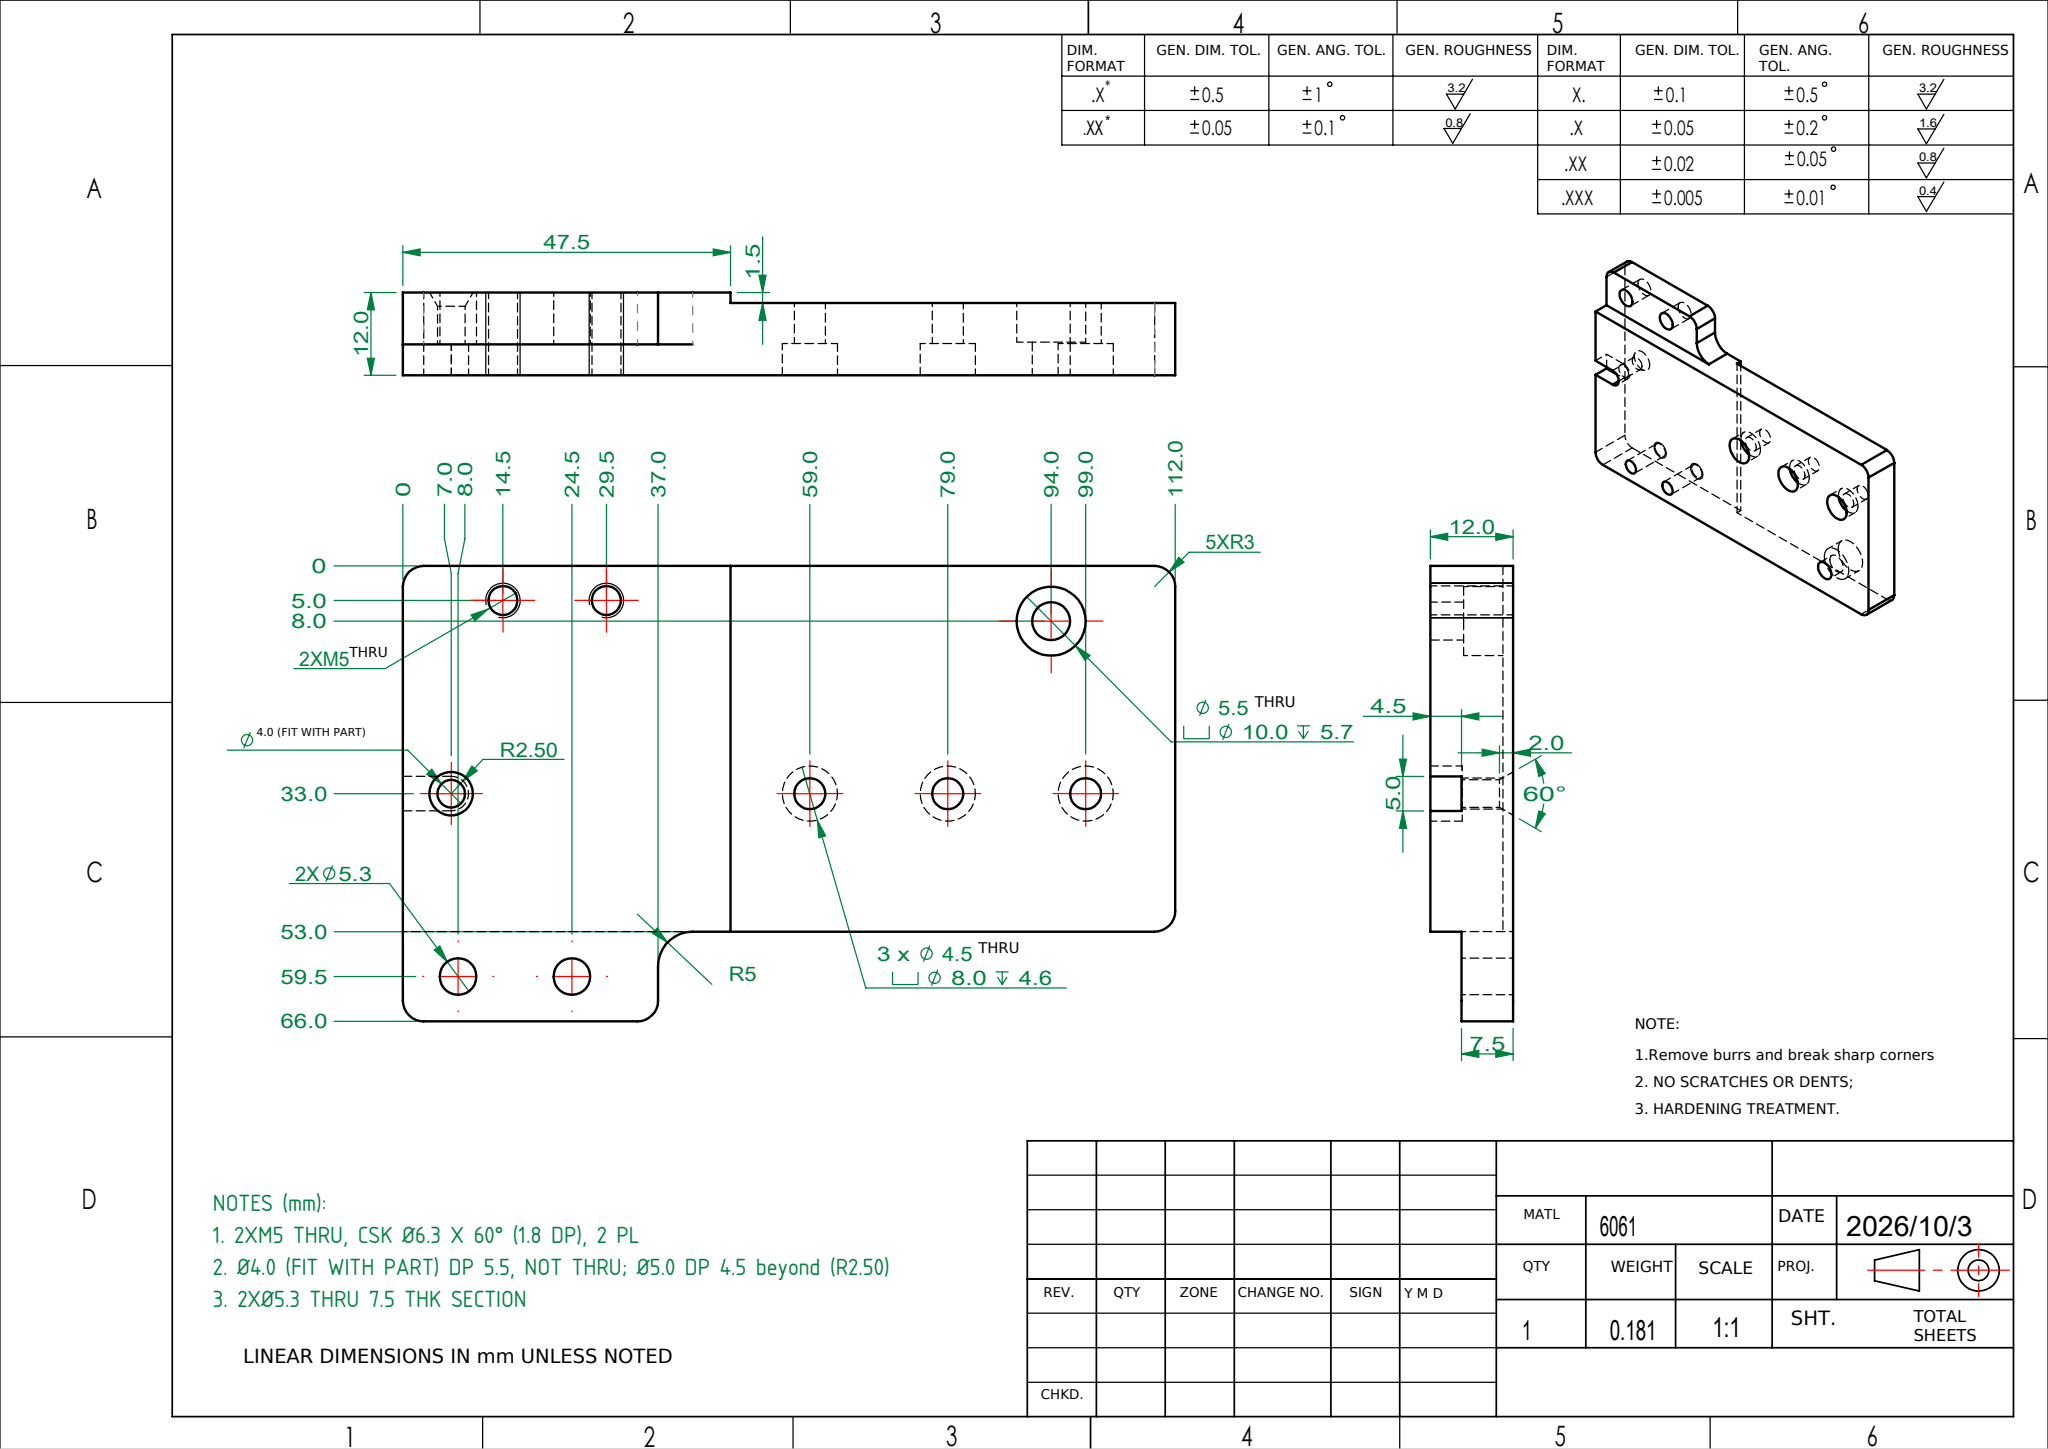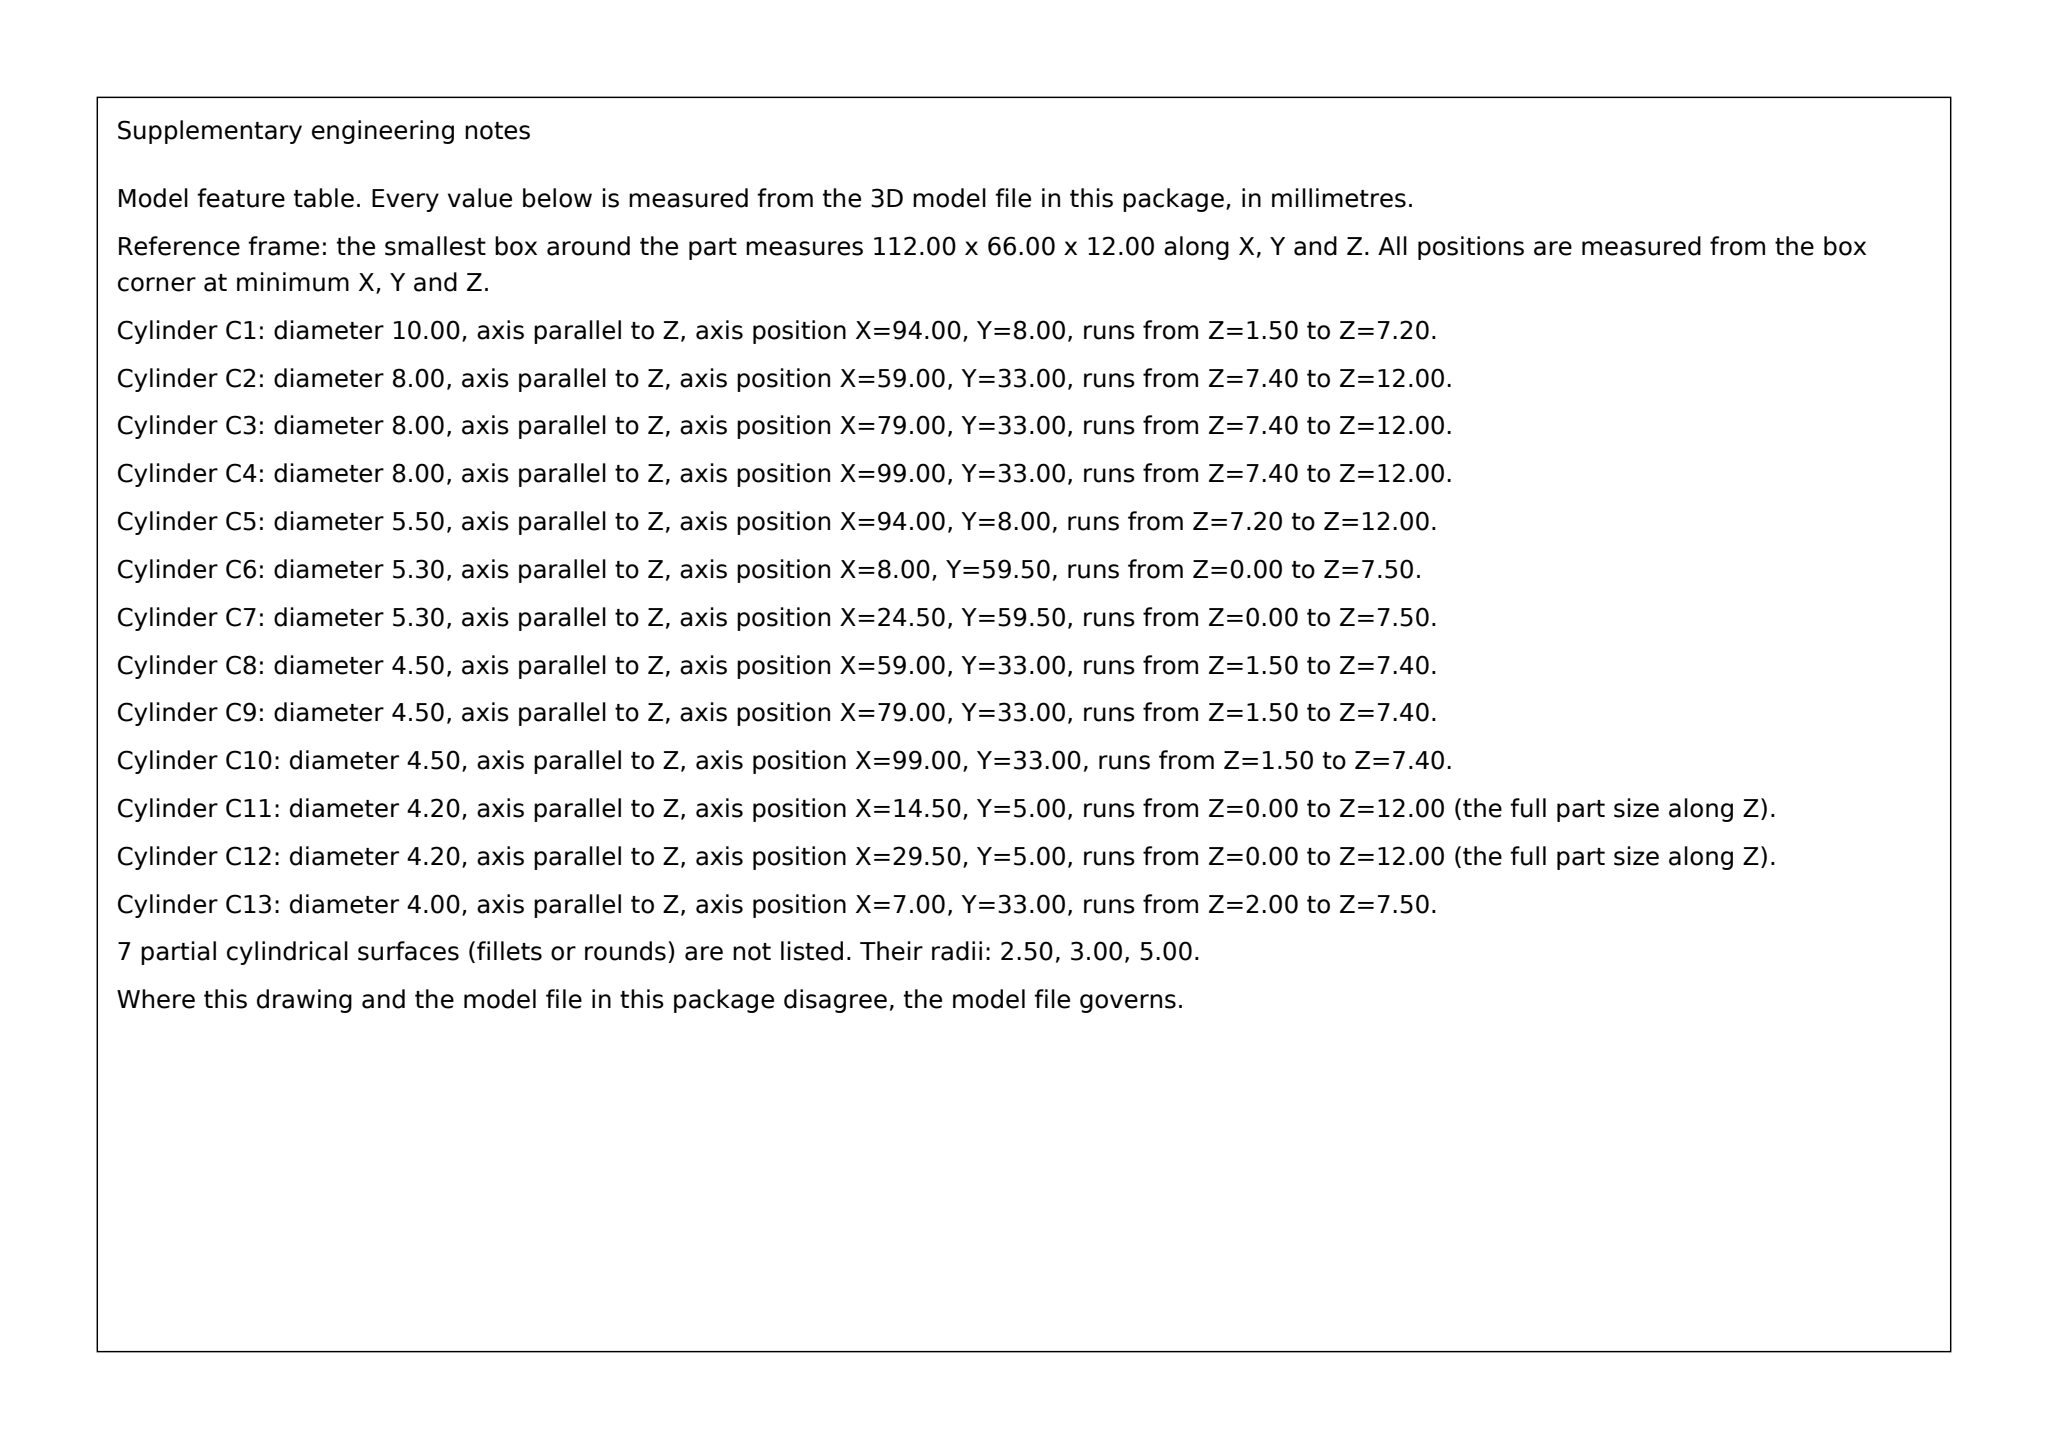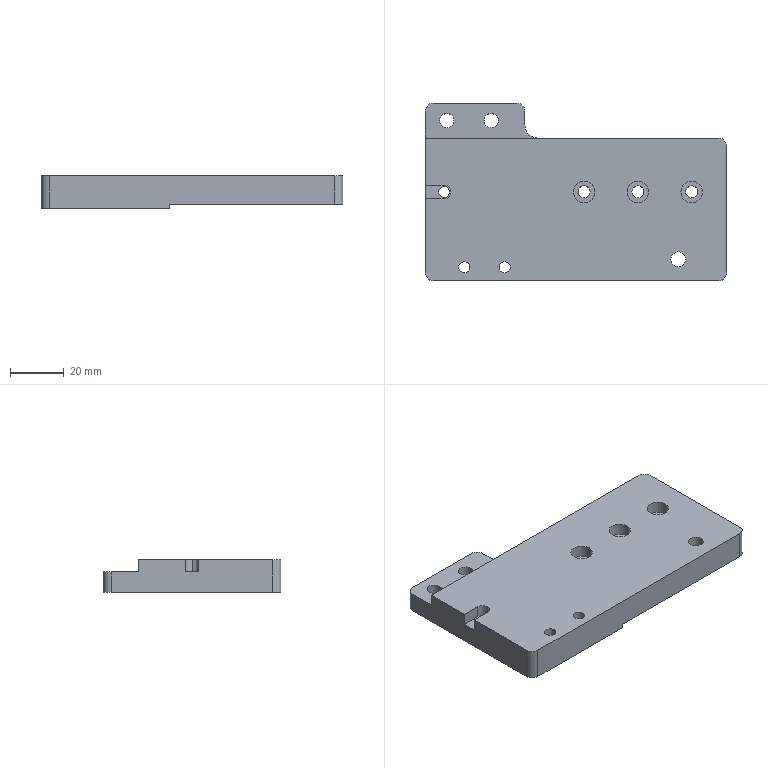Part | SolidWorks | mm | 1 solid | 54 faces | box 112 x 66 x 12 mm | volume 67146 mm3 | cylinder 34 | plane 18 | cone 2 | commonest cylinder face diameters 8 x6 4.5 x6 6 x5 4.2 x4 5.3 x4 10 x3 5.5 x2 5 x2
Drawing notes:
2XM5 THRU, CSK Ø6.3 X 60° (1.8 DP), 2 PL | from the solid: cones [60.0 incl, ref_dia 6.309, qty 2] on Ø4.2 thru holes at (14.5,5.0) & (29.5,5.0)
Ø4.0 (FIT WITH PART) DP 5.5, NOT THRU; Ø5.0 DP 4.5 beyond (R2.50) | from the solid: cylinder [4.0,z,(7.0,33.0),len 5.5] + [5.0,z,(7.0,33.0),len 4.5]; plate 12.0 thk
2XØ5.3 THRU 7.5 THK SECTION | from the solid: Ø5.3 cyls at (8.0,59.5) & (24.5,59.5), len 7.5 = local thk (z 0 to 7.5 face)
build123d program:
from build123d import *

# Parameters (mm, degrees)
SKETCH1_W                                         = 112
SKETCH1_H                                         = 66
BOSS_EXTRUDE1_DEPTH                               = 12
SKETCH2_R                                         = 2
CUT_EXTRUDE1_DEPTH                                = 32
HOLE_SIZE_ACCORDING_TO_TYPE_1_HEXAGON_D           = 4.5
HOLE_SIZE_ACCORDING_TO_TYPE_1_HEXAGON_CBORE_D     = 8
HOLE_SIZE_ACCORDING_TO_TYPE_1_HEXAGON_CBORE_DEPTH = 4.6
SKETCH5_W                                         = 64.5
SKETCH5_H                                         = 66
CUT_EXTRUDE2_DEPTH                                = 1.5
CUT_EXTRUDE3_DEPTH                                = 4.5
SKETCH7_W                                         = 112
SKETCH7_H                                         = 13
CUT_EXTRUDE4_DEPTH                                = 4.5
F_5_3_5_3_DIAMETER_HOLE1_D                        = 5.3
HOLE_SIZE_ACCORDING_TO_TYPE_3_HEXAGON_D           = 5.5
HOLE_SIZE_ACCORDING_TO_TYPE_3_HEXAGON_CBORE_D     = 10
HOLE_SIZE_ACCORDING_TO_TYPE_3_HEXAGON_CBORE_DEPTH = 5.7
M5_TAPPED_HOLE1_D                                 = 4.2
SKETCH14_W                                        = 75
SKETCH14_H                                        = 13
CUT_EXTRUDE5_DEPTH                                = 27.5
FILLET1_R                                         = 5
FILLET2_R                                         = 3
CHAMFER1_SIZE                                     = 2
CHAMFER1_SIZE2                                    = 1.155


with BuildPart() as part:
    # Sketch1 → Boss-Extrude1 (new body)
    with BuildSketch(Plane.XY):
        Rectangle(SKETCH1_W, SKETCH1_H)
    extrude(amount=BOSS_EXTRUDE1_DEPTH)

    # Sketch2 → Cut-Extrude1 (cut)
    with BuildSketch(Plane.XY.offset(12)):
        with Locations((-49, 0)):
            Circle(SKETCH2_R)
    extrude(amount=-CUT_EXTRUDE1_DEPTH, mode=Mode.SUBTRACT)

    # Hole Size _ according to_ Type 1 Hexagon (through all)
    with Locations(Plane(origin=(43, 0, 12), x_dir=(1, 0, 0), z_dir=(0, 0, 1))):
        with Locations((0, 0), (-20, 0), (-40, 0)):
            CounterBoreHole(HOLE_SIZE_ACCORDING_TO_TYPE_1_HEXAGON_D / 2, HOLE_SIZE_ACCORDING_TO_TYPE_1_HEXAGON_CBORE_D / 2, HOLE_SIZE_ACCORDING_TO_TYPE_1_HEXAGON_CBORE_DEPTH)

    # Sketch5 → Cut-Extrude2 (cut)
    with BuildSketch(Plane(origin=(0, 0, 0), x_dir=(-1, 0, 0), z_dir=(0, 0, -1))):
        with Locations((-23.75, 0)):
            Rectangle(SKETCH5_W, SKETCH5_H)
    extrude(amount=-CUT_EXTRUDE2_DEPTH, mode=Mode.SUBTRACT)

    # Sketch6 → Cut-Extrude3 (cut)
    with BuildSketch(Plane.XY.offset(12)):
        with BuildLine():
            Line((-56, 2.5), (-49, 2.5))
            ThreePointArc((-49, 2.5), (-46.5, 0), (-49, -2.5))
            Line((-49, -2.5), (-56, -2.5))
            ThreePointArc((-56, -2.5), (-58.5, 0), (-56, 2.5))
        make_face()
    extrude(amount=-CUT_EXTRUDE3_DEPTH, mode=Mode.SUBTRACT)

    # Sketch7 → Cut-Extrude4 (cut)
    with BuildSketch(Plane.XY.offset(12)):
        with Locations((0, 26.5)):
            Rectangle(SKETCH7_W, SKETCH7_H)
    extrude(amount=-CUT_EXTRUDE4_DEPTH, mode=Mode.SUBTRACT)

    # 5.3 _5.3_ Diameter Hole1 (through all)
    with Locations(Plane(origin=(-48, 26.5, 0), x_dir=(-1, 0, 0), z_dir=(0, 0, -1))):
        with Locations((0, 0), (-16.5, 0)):
            Hole(F_5_3_5_3_DIAMETER_HOLE1_D / 2)

    # Hole Size _ according to_ Type 3 Hexagon (through all)
    with Locations(Plane(origin=(38, -25, 1.5), x_dir=(-1, 0, 0), z_dir=(0, 0, -1))):
        with Locations((0, 0)):
            CounterBoreHole(HOLE_SIZE_ACCORDING_TO_TYPE_3_HEXAGON_D / 2, HOLE_SIZE_ACCORDING_TO_TYPE_3_HEXAGON_CBORE_D / 2, HOLE_SIZE_ACCORDING_TO_TYPE_3_HEXAGON_CBORE_DEPTH)

    # M5 Tapped Hole1 (through all)
    with Locations(Plane(origin=(-41.5, -28, 0), x_dir=(-1, 0, 0), z_dir=(0, 0, -1))):
        with Locations((0, 0), (-15, 0)):
            Hole(M5_TAPPED_HOLE1_D / 2)

    # Sketch14 → Cut-Extrude5 (cut)
    with BuildSketch(Plane(origin=(0, 0, 0), x_dir=(-1, 0, 0), z_dir=(0, 0, -1))):
        with Locations((-18.5, 26.5)):
            Rectangle(SKETCH14_W, SKETCH14_H)
    extrude(amount=-CUT_EXTRUDE5_DEPTH, mode=Mode.SUBTRACT)

    # Fillet1
    fillet1_edges = [part.edges().sort_by_distance(p)[0] for p in [
        (-19, 20, 3.75),
    ]]
    fillet(fillet1_edges, radius=FILLET1_R)

    # Fillet2
    fillet2_edges = [part.edges().sort_by_distance(p)[0] for p in [
        (-19, 33, 3.75),
        (56, -33, 6.75),
        (-56, -33, 6),
        (-56, 33, 3.75),
        (56, 20, 6.75),
    ]]
    fillet(fillet2_edges, radius=FILLET2_R)

    # Chamfer1
    chamfer1_edges = [part.edges().sort_by_distance(p)[0] for p in [
        (-51, 0, 0),
    ]]
    chamfer1_side = [part.faces().sort_by_distance(p)[0] for p in [
        (-51, 0, 3.75),
    ]]
    chamfer(chamfer1_edges, length=CHAMFER1_SIZE, length2=CHAMFER1_SIZE2, reference=chamfer1_side[0])


solid = part.part